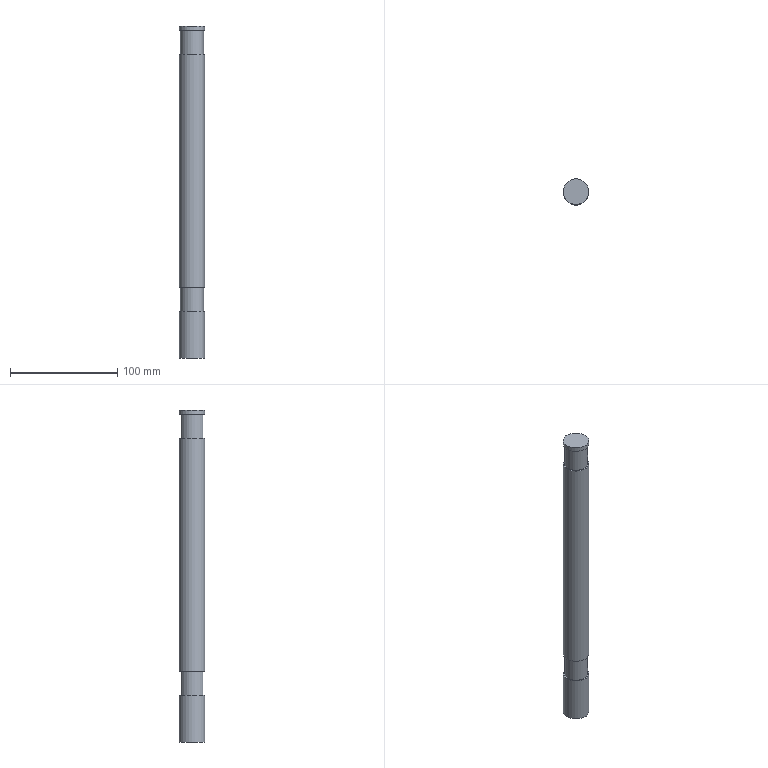Component | NX | FIX_SCREW | 1 solid | 11 faces | box 24 x 24 x 310 mm | volume 136318 mm3 | plane 6 | cylinder 5 | commonest cylinder face diameters 24 x3 21.564 x2
STEP:
#1=CARTESIAN_POINT('',(0.,0.,0.));
#2=DIRECTION('',(0.,0.,1.));
#3=DIRECTION('',(1.,0.,0.));
#4=AXIS2_PLACEMENT_3D('',#1,#2,#3);
#5=CARTESIAN_POINT('',(182.,-80.,320.));
#6=VERTEX_POINT('',#5);
#7=CARTESIAN_POINT('',(170.,-80.,320.));
#8=DIRECTION('',(0.,0.,-1.));
#9=DIRECTION('',(1.,0.,0.));
#10=AXIS2_PLACEMENT_3D('',#7,#8,#9);
#11=CIRCLE('',#10,12.);
#12=CARTESIAN_POINT('',(170.,-80.,320.));
#13=DIRECTION('',(0.,0.,1.));
#14=DIRECTION('',(1.,0.,0.));
#15=AXIS2_PLACEMENT_3D('',#12,#13,#14);
#16=PLANE('',#15);
#17=CARTESIAN_POINT('',(12.,0.));
#18=CARTESIAN_POINT('',(12.,-20.785));
#19=CARTESIAN_POINT('',(-6.,-10.392));
#20=CARTESIAN_POINT('',(-24.,-0.));
#21=CARTESIAN_POINT('',(-6.,10.392));
#22=CARTESIAN_POINT('',(12.,20.785));
#23=CARTESIAN_POINT('',(12.,0.));
#24=(BOUNDED_CURVE()B_SPLINE_CURVE(2,(#17,#18,#19,#20,#21,#22,#23),.UNSPECIFIED.,.T.,.F.)B_SPLINE_CURVE_WITH_KNOTS((1,2,2,2,2,1),(-2.094,0.,2.094,4.189,6.283,8.378),.UNSPECIFIED.)CURVE()GEOMETRIC_REPRESENTATION_ITEM()RATIONAL_B_SPLINE_CURVE((1.,0.5,1.,0.5,1.,0.5,1.))REPRESENTATION_ITEM(''));
#25=(GEOMETRIC_REPRESENTATION_CONTEXT(2)PARAMETRIC_REPRESENTATION_CONTEXT()REPRESENTATION_CONTEXT('',''));
#26=DEFINITIONAL_REPRESENTATION('',(#24),#25);
#27=PCURVE('',#16,#26);
#28=CARTESIAN_POINT('',(170.,-80.,10.));
#29=DIRECTION('',(0.,0.,1.));
#30=DIRECTION('',(1.,0.,0.));
#31=AXIS2_PLACEMENT_3D('',#28,#29,#30);
#32=CYLINDRICAL_SURFACE('',#31,12.);
#33=CARTESIAN_POINT('',(6.283,310.));
#34=DIRECTION('',(-1.,0.));
#35=VECTOR('',#34,1.);
#36=LINE('',#33,#35);
#37=(GEOMETRIC_REPRESENTATION_CONTEXT(2)PARAMETRIC_REPRESENTATION_CONTEXT()REPRESENTATION_CONTEXT('',''));
#38=DEFINITIONAL_REPRESENTATION('',(#36),#37);
#39=PCURVE('',#32,#38);
#40=SURFACE_CURVE('',#11,(#27,#39),.PCURVE_S1.);
#41=EDGE_CURVE('',#6,#6,#40,.T.);
#42=ORIENTED_EDGE('',*,*,#41,.F.);
#43=EDGE_LOOP('',(#42));
#44=FACE_BOUND('',#43,.T.);
#45=ADVANCED_FACE('',(#44),#16,.T.);
#46=CARTESIAN_POINT('',(182.,-80.,316.));
#47=VERTEX_POINT('',#46);
#48=CARTESIAN_POINT('',(170.,-80.,316.));
#49=DIRECTION('',(0.,0.,-1.));
#50=DIRECTION('',(1.,0.,0.));
#51=AXIS2_PLACEMENT_3D('',#48,#49,#50);
#52=CIRCLE('',#51,12.);
#53=CARTESIAN_POINT('',(6.283,306.));
#54=DIRECTION('',(-1.,0.));
#55=VECTOR('',#54,1.);
#56=LINE('',#53,#55);
#57=(GEOMETRIC_REPRESENTATION_CONTEXT(2)PARAMETRIC_REPRESENTATION_CONTEXT()REPRESENTATION_CONTEXT('',''));
#58=DEFINITIONAL_REPRESENTATION('',(#56),#57);
#59=PCURVE('',#32,#58);
#60=CARTESIAN_POINT('',(170.,-80.,316.));
#61=DIRECTION('',(0.,0.,1.));
#62=DIRECTION('',(1.,0.,0.));
#63=AXIS2_PLACEMENT_3D('',#60,#61,#62);
#64=PLANE('',#63);
#65=CARTESIAN_POINT('',(12.,0.));
#66=CARTESIAN_POINT('',(12.,-20.785));
#67=CARTESIAN_POINT('',(-6.,-10.392));
#68=CARTESIAN_POINT('',(-24.,-0.));
#69=CARTESIAN_POINT('',(-6.,10.392));
#70=CARTESIAN_POINT('',(12.,20.785));
#71=CARTESIAN_POINT('',(12.,0.));
#72=(BOUNDED_CURVE()B_SPLINE_CURVE(2,(#65,#66,#67,#68,#69,#70,#71),.UNSPECIFIED.,.T.,.F.)B_SPLINE_CURVE_WITH_KNOTS((1,2,2,2,2,1),(-2.094,0.,2.094,4.189,6.283,8.378),.UNSPECIFIED.)CURVE()GEOMETRIC_REPRESENTATION_ITEM()RATIONAL_B_SPLINE_CURVE((1.,0.5,1.,0.5,1.,0.5,1.))REPRESENTATION_ITEM(''));
#73=(GEOMETRIC_REPRESENTATION_CONTEXT(2)PARAMETRIC_REPRESENTATION_CONTEXT()REPRESENTATION_CONTEXT('',''));
#74=DEFINITIONAL_REPRESENTATION('',(#72),#73);
#75=PCURVE('',#64,#74);
#76=SURFACE_CURVE('',#52,(#59,#75),.PCURVE_S1.);
#77=EDGE_CURVE('',#47,#47,#76,.T.);
#78=ORIENTED_EDGE('',*,*,#77,.F.);
#79=CARTESIAN_POINT('',(182.,-80.,316.));
#80=CARTESIAN_POINT('',(182.,-80.,320.));
#81=B_SPLINE_CURVE_WITH_KNOTS('',1,(#79,#80),.UNSPECIFIED.,.F.,.F.,(2,2),(306.,310.),.PIECEWISE_BEZIER_KNOTS.);
#82=CARTESIAN_POINT('',(6.283,0.));
#83=DIRECTION('',(0.,1.));
#84=VECTOR('',#83,1.);
#85=LINE('',#82,#84);
#86=(GEOMETRIC_REPRESENTATION_CONTEXT(2)PARAMETRIC_REPRESENTATION_CONTEXT()REPRESENTATION_CONTEXT('',''));
#87=DEFINITIONAL_REPRESENTATION('',(#85),#86);
#88=PCURVE('',#32,#87);
#89=CARTESIAN_POINT('',(0.,0.));
#90=DIRECTION('',(0.,1.));
#91=VECTOR('',#90,1.);
#92=LINE('',#89,#91);
#93=(GEOMETRIC_REPRESENTATION_CONTEXT(2)PARAMETRIC_REPRESENTATION_CONTEXT()REPRESENTATION_CONTEXT('',''));
#94=DEFINITIONAL_REPRESENTATION('',(#92),#93);
#95=PCURVE('',#32,#94);
#96=SEAM_CURVE('',#81,(#88,#95),.PCURVE_S1.);
#97=EDGE_CURVE('',#47,#6,#96,.T.);
#98=ORIENTED_EDGE('',*,*,#97,.T.);
#99=ORIENTED_EDGE('',*,*,#41,.T.);
#100=ORIENTED_EDGE('',*,*,#97,.F.);
#101=EDGE_LOOP('',(#78,#98,#99,#100));
#102=FACE_BOUND('',#101,.T.);
#103=ADVANCED_FACE('',(#102),#32,.T.);
#104=CARTESIAN_POINT('',(180.782,-80.,316.));
#105=VERTEX_POINT('',#104);
#106=CARTESIAN_POINT('',(170.,-80.,316.));
#107=DIRECTION('',(0.,0.,1.));
#108=DIRECTION('',(1.,0.,0.));
#109=AXIS2_PLACEMENT_3D('',#106,#107,#108);
#110=CIRCLE('',#109,10.782);
#111=CARTESIAN_POINT('',(170.,-80.,316.));
#112=DIRECTION('',(0.,0.,-1.));
#113=DIRECTION('',(-1.,0.,0.));
#114=AXIS2_PLACEMENT_3D('',#111,#112,#113);
#115=CYLINDRICAL_SURFACE('',#114,10.782);
#116=CARTESIAN_POINT('',(9.425,0.));
#117=DIRECTION('',(-1.,0.));
#118=VECTOR('',#117,1.);
#119=LINE('',#116,#118);
#120=(GEOMETRIC_REPRESENTATION_CONTEXT(2)PARAMETRIC_REPRESENTATION_CONTEXT()REPRESENTATION_CONTEXT('',''));
#121=DEFINITIONAL_REPRESENTATION('',(#119),#120);
#122=PCURVE('',#115,#121);
#123=CARTESIAN_POINT('',(0.,0.));
#124=DIRECTION('',(1.,0.));
#125=AXIS2_PLACEMENT_2D('',#123,#124);
#126=CIRCLE('',#125,10.782);
#127=(GEOMETRIC_REPRESENTATION_CONTEXT(2)PARAMETRIC_REPRESENTATION_CONTEXT()REPRESENTATION_CONTEXT('',''));
#128=DEFINITIONAL_REPRESENTATION('',(#126),#127);
#129=PCURVE('',#64,#128);
#130=SURFACE_CURVE('',#110,(#122,#129),.PCURVE_S1.);
#131=EDGE_CURVE('',#105,#105,#130,.T.);
#132=ORIENTED_EDGE('',*,*,#131,.F.);
#133=CARTESIAN_POINT('',(180.782,-80.,293.5));
#134=VERTEX_POINT('',#133);
#135=CARTESIAN_POINT('',(180.782,-80.,316.));
#136=CARTESIAN_POINT('',(180.782,-80.,293.5));
#137=B_SPLINE_CURVE_WITH_KNOTS('',1,(#135,#136),.UNSPECIFIED.,.F.,.F.,(2,2),(0.,22.5),.PIECEWISE_BEZIER_KNOTS.);
#138=CARTESIAN_POINT('',(9.425,0.));
#139=DIRECTION('',(0.,1.));
#140=VECTOR('',#139,1.);
#141=LINE('',#138,#140);
#142=(GEOMETRIC_REPRESENTATION_CONTEXT(2)PARAMETRIC_REPRESENTATION_CONTEXT()REPRESENTATION_CONTEXT('',''));
#143=DEFINITIONAL_REPRESENTATION('',(#141),#142);
#144=PCURVE('',#115,#143);
#145=CARTESIAN_POINT('',(3.142,0.));
#146=DIRECTION('',(0.,1.));
#147=VECTOR('',#146,1.);
#148=LINE('',#145,#147);
#149=(GEOMETRIC_REPRESENTATION_CONTEXT(2)PARAMETRIC_REPRESENTATION_CONTEXT()REPRESENTATION_CONTEXT('',''));
#150=DEFINITIONAL_REPRESENTATION('',(#148),#149);
#151=PCURVE('',#115,#150);
#152=SEAM_CURVE('',#137,(#144,#151),.PCURVE_S1.);
#153=EDGE_CURVE('',#105,#134,#152,.T.);
#154=ORIENTED_EDGE('',*,*,#153,.T.);
#155=CARTESIAN_POINT('',(170.,-80.,293.5));
#156=DIRECTION('',(0.,0.,1.));
#157=DIRECTION('',(1.,0.,0.));
#158=AXIS2_PLACEMENT_3D('',#155,#156,#157);
#159=CIRCLE('',#158,10.782);
#160=CARTESIAN_POINT('',(9.425,22.5));
#161=DIRECTION('',(-1.,0.));
#162=VECTOR('',#161,1.);
#163=LINE('',#160,#162);
#164=(GEOMETRIC_REPRESENTATION_CONTEXT(2)PARAMETRIC_REPRESENTATION_CONTEXT()REPRESENTATION_CONTEXT('',''));
#165=DEFINITIONAL_REPRESENTATION('',(#163),#164);
#166=PCURVE('',#115,#165);
#167=CARTESIAN_POINT('',(170.,-80.,293.5));
#168=DIRECTION('',(0.,0.,1.));
#169=DIRECTION('',(1.,0.,0.));
#170=AXIS2_PLACEMENT_3D('',#167,#168,#169);
#171=PLANE('',#170);
#172=CARTESIAN_POINT('',(0.,0.));
#173=DIRECTION('',(1.,0.));
#174=AXIS2_PLACEMENT_2D('',#172,#173);
#175=CIRCLE('',#174,10.782);
#176=(GEOMETRIC_REPRESENTATION_CONTEXT(2)PARAMETRIC_REPRESENTATION_CONTEXT()REPRESENTATION_CONTEXT('',''));
#177=DEFINITIONAL_REPRESENTATION('',(#175),#176);
#178=PCURVE('',#171,#177);
#179=SURFACE_CURVE('',#159,(#166,#178),.PCURVE_S1.);
#180=EDGE_CURVE('',#134,#134,#179,.T.);
#181=ORIENTED_EDGE('',*,*,#180,.T.);
#182=ORIENTED_EDGE('',*,*,#153,.F.);
#183=EDGE_LOOP('',(#132,#154,#181,#182));
#184=FACE_BOUND('',#183,.T.);
#185=ADVANCED_FACE('',(#184),#115,.T.);
#186=ORIENTED_EDGE('',*,*,#77,.T.);
#187=EDGE_LOOP('',(#186));
#188=FACE_BOUND('',#187,.T.);
#189=ORIENTED_EDGE('',*,*,#131,.T.);
#190=EDGE_LOOP('',(#189));
#191=FACE_BOUND('',#190,.T.);
#192=ADVANCED_FACE('',(#188,#191),#64,.F.);
#193=CARTESIAN_POINT('',(182.,-80.,293.5));
#194=VERTEX_POINT('',#193);
#195=CARTESIAN_POINT('',(170.,-80.,293.5));
#196=DIRECTION('',(0.,0.,-1.));
#197=DIRECTION('',(1.,0.,0.));
#198=AXIS2_PLACEMENT_3D('',#195,#196,#197);
#199=CIRCLE('',#198,12.);
#200=CARTESIAN_POINT('',(12.,0.));
#201=CARTESIAN_POINT('',(12.,-20.785));
#202=CARTESIAN_POINT('',(-6.,-10.392));
#203=CARTESIAN_POINT('',(-24.,-0.));
#204=CARTESIAN_POINT('',(-6.,10.392));
#205=CARTESIAN_POINT('',(12.,20.785));
#206=CARTESIAN_POINT('',(12.,0.));
#207=(BOUNDED_CURVE()B_SPLINE_CURVE(2,(#200,#201,#202,#203,#204,#205,#206),.UNSPECIFIED.,.T.,.F.)B_SPLINE_CURVE_WITH_KNOTS((1,2,2,2,2,1),(-2.094,0.,2.094,4.189,6.283,8.378),.UNSPECIFIED.)CURVE()GEOMETRIC_REPRESENTATION_ITEM()RATIONAL_B_SPLINE_CURVE((1.,0.5,1.,0.5,1.,0.5,1.))REPRESENTATION_ITEM(''));
#208=(GEOMETRIC_REPRESENTATION_CONTEXT(2)PARAMETRIC_REPRESENTATION_CONTEXT()REPRESENTATION_CONTEXT('',''));
#209=DEFINITIONAL_REPRESENTATION('',(#207),#208);
#210=PCURVE('',#171,#209);
#211=CARTESIAN_POINT('',(170.,-80.,10.));
#212=DIRECTION('',(0.,0.,1.));
#213=DIRECTION('',(1.,0.,0.));
#214=AXIS2_PLACEMENT_3D('',#211,#212,#213);
#215=CYLINDRICAL_SURFACE('',#214,12.);
#216=CARTESIAN_POINT('',(6.283,283.5));
#217=DIRECTION('',(-1.,0.));
#218=VECTOR('',#217,1.);
#219=LINE('',#216,#218);
#220=(GEOMETRIC_REPRESENTATION_CONTEXT(2)PARAMETRIC_REPRESENTATION_CONTEXT()REPRESENTATION_CONTEXT('',''));
#221=DEFINITIONAL_REPRESENTATION('',(#219),#220);
#222=PCURVE('',#215,#221);
#223=SURFACE_CURVE('',#199,(#210,#222),.PCURVE_S1.);
#224=EDGE_CURVE('',#194,#194,#223,.T.);
#225=ORIENTED_EDGE('',*,*,#224,.F.);
#226=EDGE_LOOP('',(#225));
#227=FACE_BOUND('',#226,.T.);
#228=ORIENTED_EDGE('',*,*,#180,.F.);
#229=EDGE_LOOP('',(#228));
#230=FACE_BOUND('',#229,.T.);
#231=ADVANCED_FACE('',(#227,#230),#171,.T.);
#232=CARTESIAN_POINT('',(182.,-80.,76.));
#233=VERTEX_POINT('',#232);
#234=CARTESIAN_POINT('',(170.,-80.,76.));
#235=DIRECTION('',(0.,0.,-1.));
#236=DIRECTION('',(1.,0.,0.));
#237=AXIS2_PLACEMENT_3D('',#234,#235,#236);
#238=CIRCLE('',#237,12.);
#239=CARTESIAN_POINT('',(6.283,66.));
#240=DIRECTION('',(-1.,0.));
#241=VECTOR('',#240,1.);
#242=LINE('',#239,#241);
#243=(GEOMETRIC_REPRESENTATION_CONTEXT(2)PARAMETRIC_REPRESENTATION_CONTEXT()REPRESENTATION_CONTEXT('',''));
#244=DEFINITIONAL_REPRESENTATION('',(#242),#243);
#245=PCURVE('',#215,#244);
#246=CARTESIAN_POINT('',(170.,-80.,76.));
#247=DIRECTION('',(0.,0.,1.));
#248=DIRECTION('',(1.,0.,0.));
#249=AXIS2_PLACEMENT_3D('',#246,#247,#248);
#250=PLANE('',#249);
#251=CARTESIAN_POINT('',(12.,0.));
#252=CARTESIAN_POINT('',(12.,-20.785));
#253=CARTESIAN_POINT('',(-6.,-10.392));
#254=CARTESIAN_POINT('',(-24.,-0.));
#255=CARTESIAN_POINT('',(-6.,10.392));
#256=CARTESIAN_POINT('',(12.,20.785));
#257=CARTESIAN_POINT('',(12.,0.));
#258=(BOUNDED_CURVE()B_SPLINE_CURVE(2,(#251,#252,#253,#254,#255,#256,#257),.UNSPECIFIED.,.T.,.F.)B_SPLINE_CURVE_WITH_KNOTS((1,2,2,2,2,1),(-2.094,0.,2.094,4.189,6.283,8.378),.UNSPECIFIED.)CURVE()GEOMETRIC_REPRESENTATION_ITEM()RATIONAL_B_SPLINE_CURVE((1.,0.5,1.,0.5,1.,0.5,1.))REPRESENTATION_ITEM(''));
#259=(GEOMETRIC_REPRESENTATION_CONTEXT(2)PARAMETRIC_REPRESENTATION_CONTEXT()REPRESENTATION_CONTEXT('',''));
#260=DEFINITIONAL_REPRESENTATION('',(#258),#259);
#261=PCURVE('',#250,#260);
#262=SURFACE_CURVE('',#238,(#245,#261),.PCURVE_S1.);
#263=EDGE_CURVE('',#233,#233,#262,.T.);
#264=ORIENTED_EDGE('',*,*,#263,.F.);
#265=CARTESIAN_POINT('',(182.,-80.,76.));
#266=CARTESIAN_POINT('',(182.,-80.,293.5));
#267=B_SPLINE_CURVE_WITH_KNOTS('',1,(#265,#266),.UNSPECIFIED.,.F.,.F.,(2,2),(66.,283.5),.PIECEWISE_BEZIER_KNOTS.);
#268=CARTESIAN_POINT('',(6.283,0.));
#269=DIRECTION('',(0.,1.));
#270=VECTOR('',#269,1.);
#271=LINE('',#268,#270);
#272=(GEOMETRIC_REPRESENTATION_CONTEXT(2)PARAMETRIC_REPRESENTATION_CONTEXT()REPRESENTATION_CONTEXT('',''));
#273=DEFINITIONAL_REPRESENTATION('',(#271),#272);
#274=PCURVE('',#215,#273);
#275=CARTESIAN_POINT('',(0.,0.));
#276=DIRECTION('',(0.,1.));
#277=VECTOR('',#276,1.);
#278=LINE('',#275,#277);
#279=(GEOMETRIC_REPRESENTATION_CONTEXT(2)PARAMETRIC_REPRESENTATION_CONTEXT()REPRESENTATION_CONTEXT('',''));
#280=DEFINITIONAL_REPRESENTATION('',(#278),#279);
#281=PCURVE('',#215,#280);
#282=SEAM_CURVE('',#267,(#274,#281),.PCURVE_S1.);
#283=EDGE_CURVE('',#233,#194,#282,.T.);
#284=ORIENTED_EDGE('',*,*,#283,.T.);
#285=ORIENTED_EDGE('',*,*,#224,.T.);
#286=ORIENTED_EDGE('',*,*,#283,.F.);
#287=EDGE_LOOP('',(#264,#284,#285,#286));
#288=FACE_BOUND('',#287,.T.);
#289=ADVANCED_FACE('',(#288),#215,.T.);
#290=CARTESIAN_POINT('',(180.782,-80.,76.));
#291=VERTEX_POINT('',#290);
#292=CARTESIAN_POINT('',(170.,-80.,76.));
#293=DIRECTION('',(0.,0.,1.));
#294=DIRECTION('',(1.,0.,0.));
#295=AXIS2_PLACEMENT_3D('',#292,#293,#294);
#296=CIRCLE('',#295,10.782);
#297=CARTESIAN_POINT('',(170.,-80.,76.));
#298=DIRECTION('',(0.,0.,-1.));
#299=DIRECTION('',(-1.,0.,0.));
#300=AXIS2_PLACEMENT_3D('',#297,#298,#299);
#301=CYLINDRICAL_SURFACE('',#300,10.782);
#302=CARTESIAN_POINT('',(9.425,0.));
#303=DIRECTION('',(-1.,0.));
#304=VECTOR('',#303,1.);
#305=LINE('',#302,#304);
#306=(GEOMETRIC_REPRESENTATION_CONTEXT(2)PARAMETRIC_REPRESENTATION_CONTEXT()REPRESENTATION_CONTEXT('',''));
#307=DEFINITIONAL_REPRESENTATION('',(#305),#306);
#308=PCURVE('',#301,#307);
#309=CARTESIAN_POINT('',(0.,0.));
#310=DIRECTION('',(1.,0.));
#311=AXIS2_PLACEMENT_2D('',#309,#310);
#312=CIRCLE('',#311,10.782);
#313=(GEOMETRIC_REPRESENTATION_CONTEXT(2)PARAMETRIC_REPRESENTATION_CONTEXT()REPRESENTATION_CONTEXT('',''));
#314=DEFINITIONAL_REPRESENTATION('',(#312),#313);
#315=PCURVE('',#250,#314);
#316=SURFACE_CURVE('',#296,(#308,#315),.PCURVE_S1.);
#317=EDGE_CURVE('',#291,#291,#316,.T.);
#318=ORIENTED_EDGE('',*,*,#317,.F.);
#319=CARTESIAN_POINT('',(180.782,-80.,53.5));
#320=VERTEX_POINT('',#319);
#321=CARTESIAN_POINT('',(180.782,-80.,76.));
#322=CARTESIAN_POINT('',(180.782,-80.,53.5));
#323=B_SPLINE_CURVE_WITH_KNOTS('',1,(#321,#322),.UNSPECIFIED.,.F.,.F.,(2,2),(0.,22.5),.PIECEWISE_BEZIER_KNOTS.);
#324=CARTESIAN_POINT('',(9.425,0.));
#325=DIRECTION('',(0.,1.));
#326=VECTOR('',#325,1.);
#327=LINE('',#324,#326);
#328=(GEOMETRIC_REPRESENTATION_CONTEXT(2)PARAMETRIC_REPRESENTATION_CONTEXT()REPRESENTATION_CONTEXT('',''));
#329=DEFINITIONAL_REPRESENTATION('',(#327),#328);
#330=PCURVE('',#301,#329);
#331=CARTESIAN_POINT('',(3.142,0.));
#332=DIRECTION('',(0.,1.));
#333=VECTOR('',#332,1.);
#334=LINE('',#331,#333);
#335=(GEOMETRIC_REPRESENTATION_CONTEXT(2)PARAMETRIC_REPRESENTATION_CONTEXT()REPRESENTATION_CONTEXT('',''));
#336=DEFINITIONAL_REPRESENTATION('',(#334),#335);
#337=PCURVE('',#301,#336);
#338=SEAM_CURVE('',#323,(#330,#337),.PCURVE_S1.);
#339=EDGE_CURVE('',#291,#320,#338,.T.);
#340=ORIENTED_EDGE('',*,*,#339,.T.);
#341=CARTESIAN_POINT('',(170.,-80.,53.5));
#342=DIRECTION('',(0.,0.,1.));
#343=DIRECTION('',(1.,0.,0.));
#344=AXIS2_PLACEMENT_3D('',#341,#342,#343);
#345=CIRCLE('',#344,10.782);
#346=CARTESIAN_POINT('',(9.425,22.5));
#347=DIRECTION('',(-1.,0.));
#348=VECTOR('',#347,1.);
#349=LINE('',#346,#348);
#350=(GEOMETRIC_REPRESENTATION_CONTEXT(2)PARAMETRIC_REPRESENTATION_CONTEXT()REPRESENTATION_CONTEXT('',''));
#351=DEFINITIONAL_REPRESENTATION('',(#349),#350);
#352=PCURVE('',#301,#351);
#353=CARTESIAN_POINT('',(170.,-80.,53.5));
#354=DIRECTION('',(0.,0.,1.));
#355=DIRECTION('',(1.,0.,0.));
#356=AXIS2_PLACEMENT_3D('',#353,#354,#355);
#357=PLANE('',#356);
#358=CARTESIAN_POINT('',(0.,0.));
#359=DIRECTION('',(1.,0.));
#360=AXIS2_PLACEMENT_2D('',#358,#359);
#361=CIRCLE('',#360,10.782);
#362=(GEOMETRIC_REPRESENTATION_CONTEXT(2)PARAMETRIC_REPRESENTATION_CONTEXT()REPRESENTATION_CONTEXT('',''));
#363=DEFINITIONAL_REPRESENTATION('',(#361),#362);
#364=PCURVE('',#357,#363);
#365=SURFACE_CURVE('',#345,(#352,#364),.PCURVE_S1.);
#366=EDGE_CURVE('',#320,#320,#365,.T.);
#367=ORIENTED_EDGE('',*,*,#366,.T.);
#368=ORIENTED_EDGE('',*,*,#339,.F.);
#369=EDGE_LOOP('',(#318,#340,#367,#368));
#370=FACE_BOUND('',#369,.T.);
#371=ADVANCED_FACE('',(#370),#301,.T.);
#372=ORIENTED_EDGE('',*,*,#263,.T.);
#373=EDGE_LOOP('',(#372));
#374=FACE_BOUND('',#373,.T.);
#375=ORIENTED_EDGE('',*,*,#317,.T.);
#376=EDGE_LOOP('',(#375));
#377=FACE_BOUND('',#376,.T.);
#378=ADVANCED_FACE('',(#374,#377),#250,.F.);
#379=CARTESIAN_POINT('',(182.,-80.,53.5));
#380=VERTEX_POINT('',#379);
#381=CARTESIAN_POINT('',(170.,-80.,53.5));
#382=DIRECTION('',(0.,0.,-1.));
#383=DIRECTION('',(1.,0.,0.));
#384=AXIS2_PLACEMENT_3D('',#381,#382,#383);
#385=CIRCLE('',#384,12.);
#386=CARTESIAN_POINT('',(12.,0.));
#387=CARTESIAN_POINT('',(12.,-20.785));
#388=CARTESIAN_POINT('',(-6.,-10.392));
#389=CARTESIAN_POINT('',(-24.,-0.));
#390=CARTESIAN_POINT('',(-6.,10.392));
#391=CARTESIAN_POINT('',(12.,20.785));
#392=CARTESIAN_POINT('',(12.,0.));
#393=(BOUNDED_CURVE()B_SPLINE_CURVE(2,(#386,#387,#388,#389,#390,#391,#392),.UNSPECIFIED.,.T.,.F.)B_SPLINE_CURVE_WITH_KNOTS((1,2,2,2,2,1),(-2.094,0.,2.094,4.189,6.283,8.378),.UNSPECIFIED.)CURVE()GEOMETRIC_REPRESENTATION_ITEM()RATIONAL_B_SPLINE_CURVE((1.,0.5,1.,0.5,1.,0.5,1.))REPRESENTATION_ITEM(''));
#394=(GEOMETRIC_REPRESENTATION_CONTEXT(2)PARAMETRIC_REPRESENTATION_CONTEXT()REPRESENTATION_CONTEXT('',''));
#395=DEFINITIONAL_REPRESENTATION('',(#393),#394);
#396=PCURVE('',#357,#395);
#397=CARTESIAN_POINT('',(170.,-80.,10.));
#398=DIRECTION('',(0.,0.,1.));
#399=DIRECTION('',(1.,0.,0.));
#400=AXIS2_PLACEMENT_3D('',#397,#398,#399);
#401=CYLINDRICAL_SURFACE('',#400,12.);
#402=CARTESIAN_POINT('',(6.283,43.5));
#403=DIRECTION('',(-1.,0.));
#404=VECTOR('',#403,1.);
#405=LINE('',#402,#404);
#406=(GEOMETRIC_REPRESENTATION_CONTEXT(2)PARAMETRIC_REPRESENTATION_CONTEXT()REPRESENTATION_CONTEXT('',''));
#407=DEFINITIONAL_REPRESENTATION('',(#405),#406);
#408=PCURVE('',#401,#407);
#409=SURFACE_CURVE('',#385,(#396,#408),.PCURVE_S1.);
#410=EDGE_CURVE('',#380,#380,#409,.T.);
#411=ORIENTED_EDGE('',*,*,#410,.F.);
#412=EDGE_LOOP('',(#411));
#413=FACE_BOUND('',#412,.T.);
#414=ORIENTED_EDGE('',*,*,#366,.F.);
#415=EDGE_LOOP('',(#414));
#416=FACE_BOUND('',#415,.T.);
#417=ADVANCED_FACE('',(#413,#416),#357,.T.);
#418=CARTESIAN_POINT('',(182.,-80.,10.));
#419=VERTEX_POINT('',#418);
#420=CARTESIAN_POINT('',(170.,-80.,10.));
#421=DIRECTION('',(0.,0.,1.));
#422=DIRECTION('',(1.,0.,0.));
#423=AXIS2_PLACEMENT_3D('',#420,#421,#422);
#424=CIRCLE('',#423,12.);
#425=CARTESIAN_POINT('',(170.,-80.,10.));
#426=DIRECTION('',(0.,0.,-1.));
#427=DIRECTION('',(-1.,0.,0.));
#428=AXIS2_PLACEMENT_3D('',#425,#426,#427);
#429=PLANE('',#428);
#430=CARTESIAN_POINT('',(-12.,0.));
#431=CARTESIAN_POINT('',(-12.,20.785));
#432=CARTESIAN_POINT('',(6.,10.392));
#433=CARTESIAN_POINT('',(24.,0.));
#434=CARTESIAN_POINT('',(6.,-10.392));
#435=CARTESIAN_POINT('',(-12.,-20.785));
#436=CARTESIAN_POINT('',(-12.,0.));
#437=(BOUNDED_CURVE()B_SPLINE_CURVE(2,(#430,#431,#432,#433,#434,#435,#436),.UNSPECIFIED.,.T.,.F.)B_SPLINE_CURVE_WITH_KNOTS((1,2,2,2,2,1),(-2.094,0.,2.094,4.189,6.283,8.378),.UNSPECIFIED.)CURVE()GEOMETRIC_REPRESENTATION_ITEM()RATIONAL_B_SPLINE_CURVE((1.,0.5,1.,0.5,1.,0.5,1.))REPRESENTATION_ITEM(''));
#438=(GEOMETRIC_REPRESENTATION_CONTEXT(2)PARAMETRIC_REPRESENTATION_CONTEXT()REPRESENTATION_CONTEXT('',''));
#439=DEFINITIONAL_REPRESENTATION('',(#437),#438);
#440=PCURVE('',#429,#439);
#441=CARTESIAN_POINT('',(0.,0.));
#442=DIRECTION('',(1.,0.));
#443=VECTOR('',#442,1.);
#444=LINE('',#441,#443);
#445=(GEOMETRIC_REPRESENTATION_CONTEXT(2)PARAMETRIC_REPRESENTATION_CONTEXT()REPRESENTATION_CONTEXT('',''));
#446=DEFINITIONAL_REPRESENTATION('',(#444),#445);
#447=PCURVE('',#401,#446);
#448=SURFACE_CURVE('',#424,(#440,#447),.PCURVE_S1.);
#449=EDGE_CURVE('',#419,#419,#448,.T.);
#450=ORIENTED_EDGE('',*,*,#449,.F.);
#451=EDGE_LOOP('',(#450));
#452=FACE_BOUND('',#451,.T.);
#453=ADVANCED_FACE('',(#452),#429,.T.);
#454=ORIENTED_EDGE('',*,*,#449,.T.);
#455=CARTESIAN_POINT('',(182.,-80.,10.));
#456=CARTESIAN_POINT('',(182.,-80.,53.5));
#457=B_SPLINE_CURVE_WITH_KNOTS('',1,(#455,#456),.UNSPECIFIED.,.F.,.F.,(2,2),(0.,43.5),.PIECEWISE_BEZIER_KNOTS.);
#458=CARTESIAN_POINT('',(6.283,0.));
#459=DIRECTION('',(0.,1.));
#460=VECTOR('',#459,1.);
#461=LINE('',#458,#460);
#462=(GEOMETRIC_REPRESENTATION_CONTEXT(2)PARAMETRIC_REPRESENTATION_CONTEXT()REPRESENTATION_CONTEXT('',''));
#463=DEFINITIONAL_REPRESENTATION('',(#461),#462);
#464=PCURVE('',#401,#463);
#465=CARTESIAN_POINT('',(0.,0.));
#466=DIRECTION('',(0.,1.));
#467=VECTOR('',#466,1.);
#468=LINE('',#465,#467);
#469=(GEOMETRIC_REPRESENTATION_CONTEXT(2)PARAMETRIC_REPRESENTATION_CONTEXT()REPRESENTATION_CONTEXT('',''));
#470=DEFINITIONAL_REPRESENTATION('',(#468),#469);
#471=PCURVE('',#401,#470);
#472=SEAM_CURVE('',#457,(#464,#471),.PCURVE_S1.);
#473=EDGE_CURVE('',#419,#380,#472,.T.);
#474=ORIENTED_EDGE('',*,*,#473,.T.);
#475=ORIENTED_EDGE('',*,*,#410,.T.);
#476=ORIENTED_EDGE('',*,*,#473,.F.);
#477=EDGE_LOOP('',(#454,#474,#475,#476));
#478=FACE_BOUND('',#477,.T.);
#479=ADVANCED_FACE('',(#478),#401,.T.);
#480=CLOSED_SHELL('',(#45,#103,#185,#192,#231,#289,#371,#378,#417,#453,#479));
#481=MANIFOLD_SOLID_BREP('',#480);
#482=(LENGTH_UNIT()NAMED_UNIT(*)SI_UNIT(.MILLI.,.METRE.));
#483=UNCERTAINTY_MEASURE_WITH_UNIT(LENGTH_MEASURE(0.00001),#482,'','');
#484=(NAMED_UNIT(*)PLANE_ANGLE_UNIT()SI_UNIT($,.RADIAN.));
#485=(NAMED_UNIT(*)SI_UNIT($,.STERADIAN.)SOLID_ANGLE_UNIT());
#486=(GEOMETRIC_REPRESENTATION_CONTEXT(3)GLOBAL_UNCERTAINTY_ASSIGNED_CONTEXT((#483))GLOBAL_UNIT_ASSIGNED_CONTEXT((#482,#484,#485))REPRESENTATION_CONTEXT('',''));
#487=ADVANCED_BREP_SHAPE_REPRESENTATION('',(#4,#481),#486);